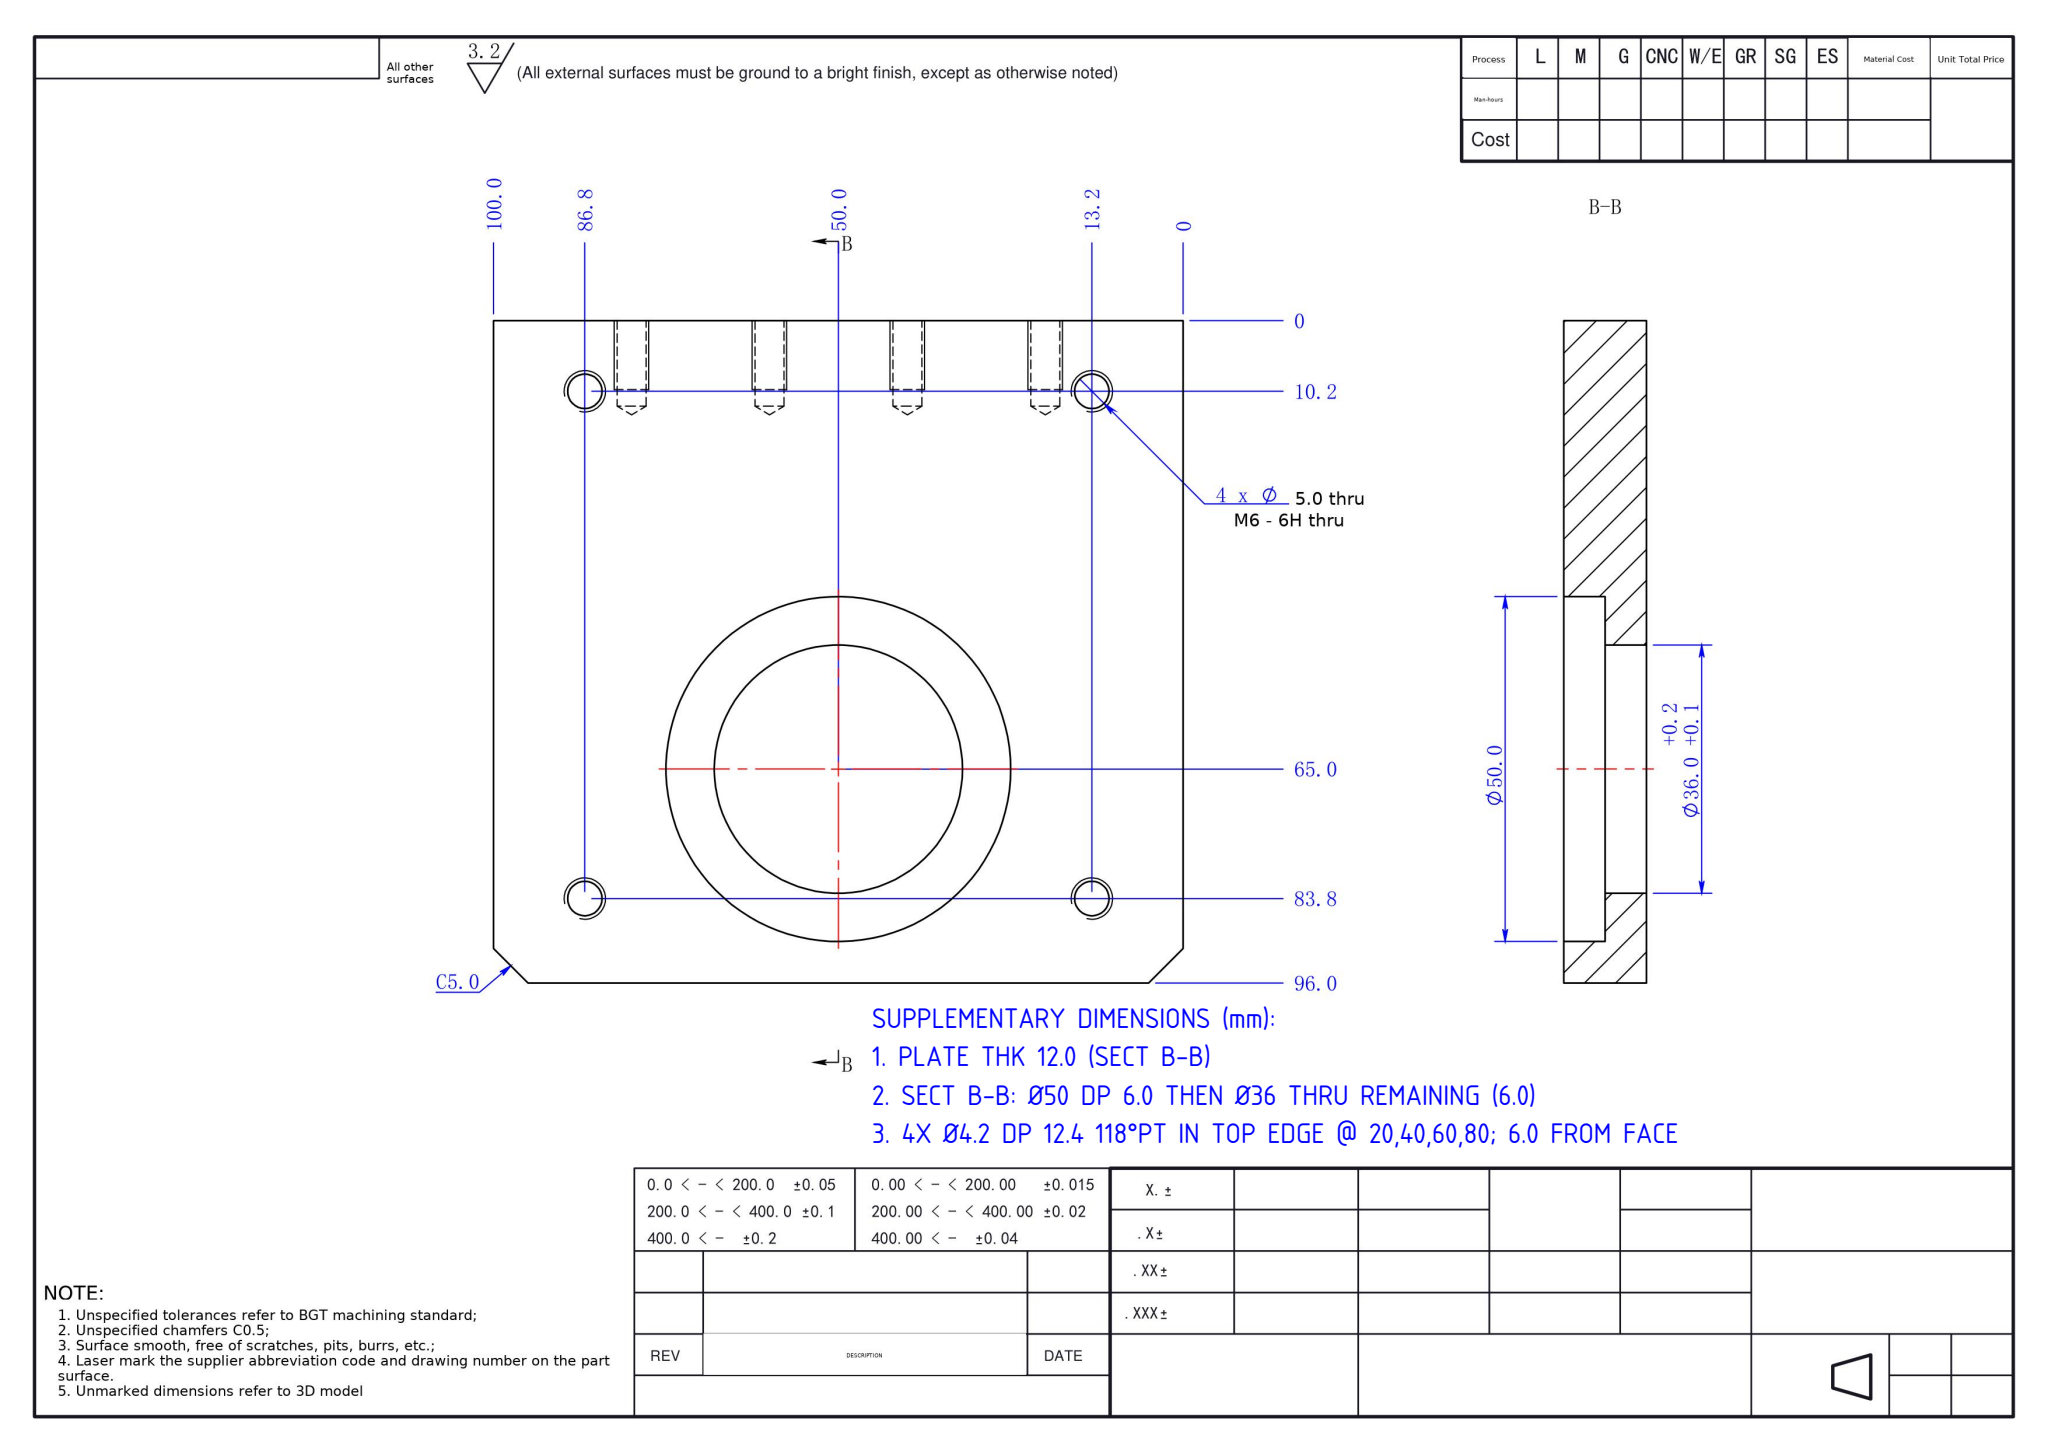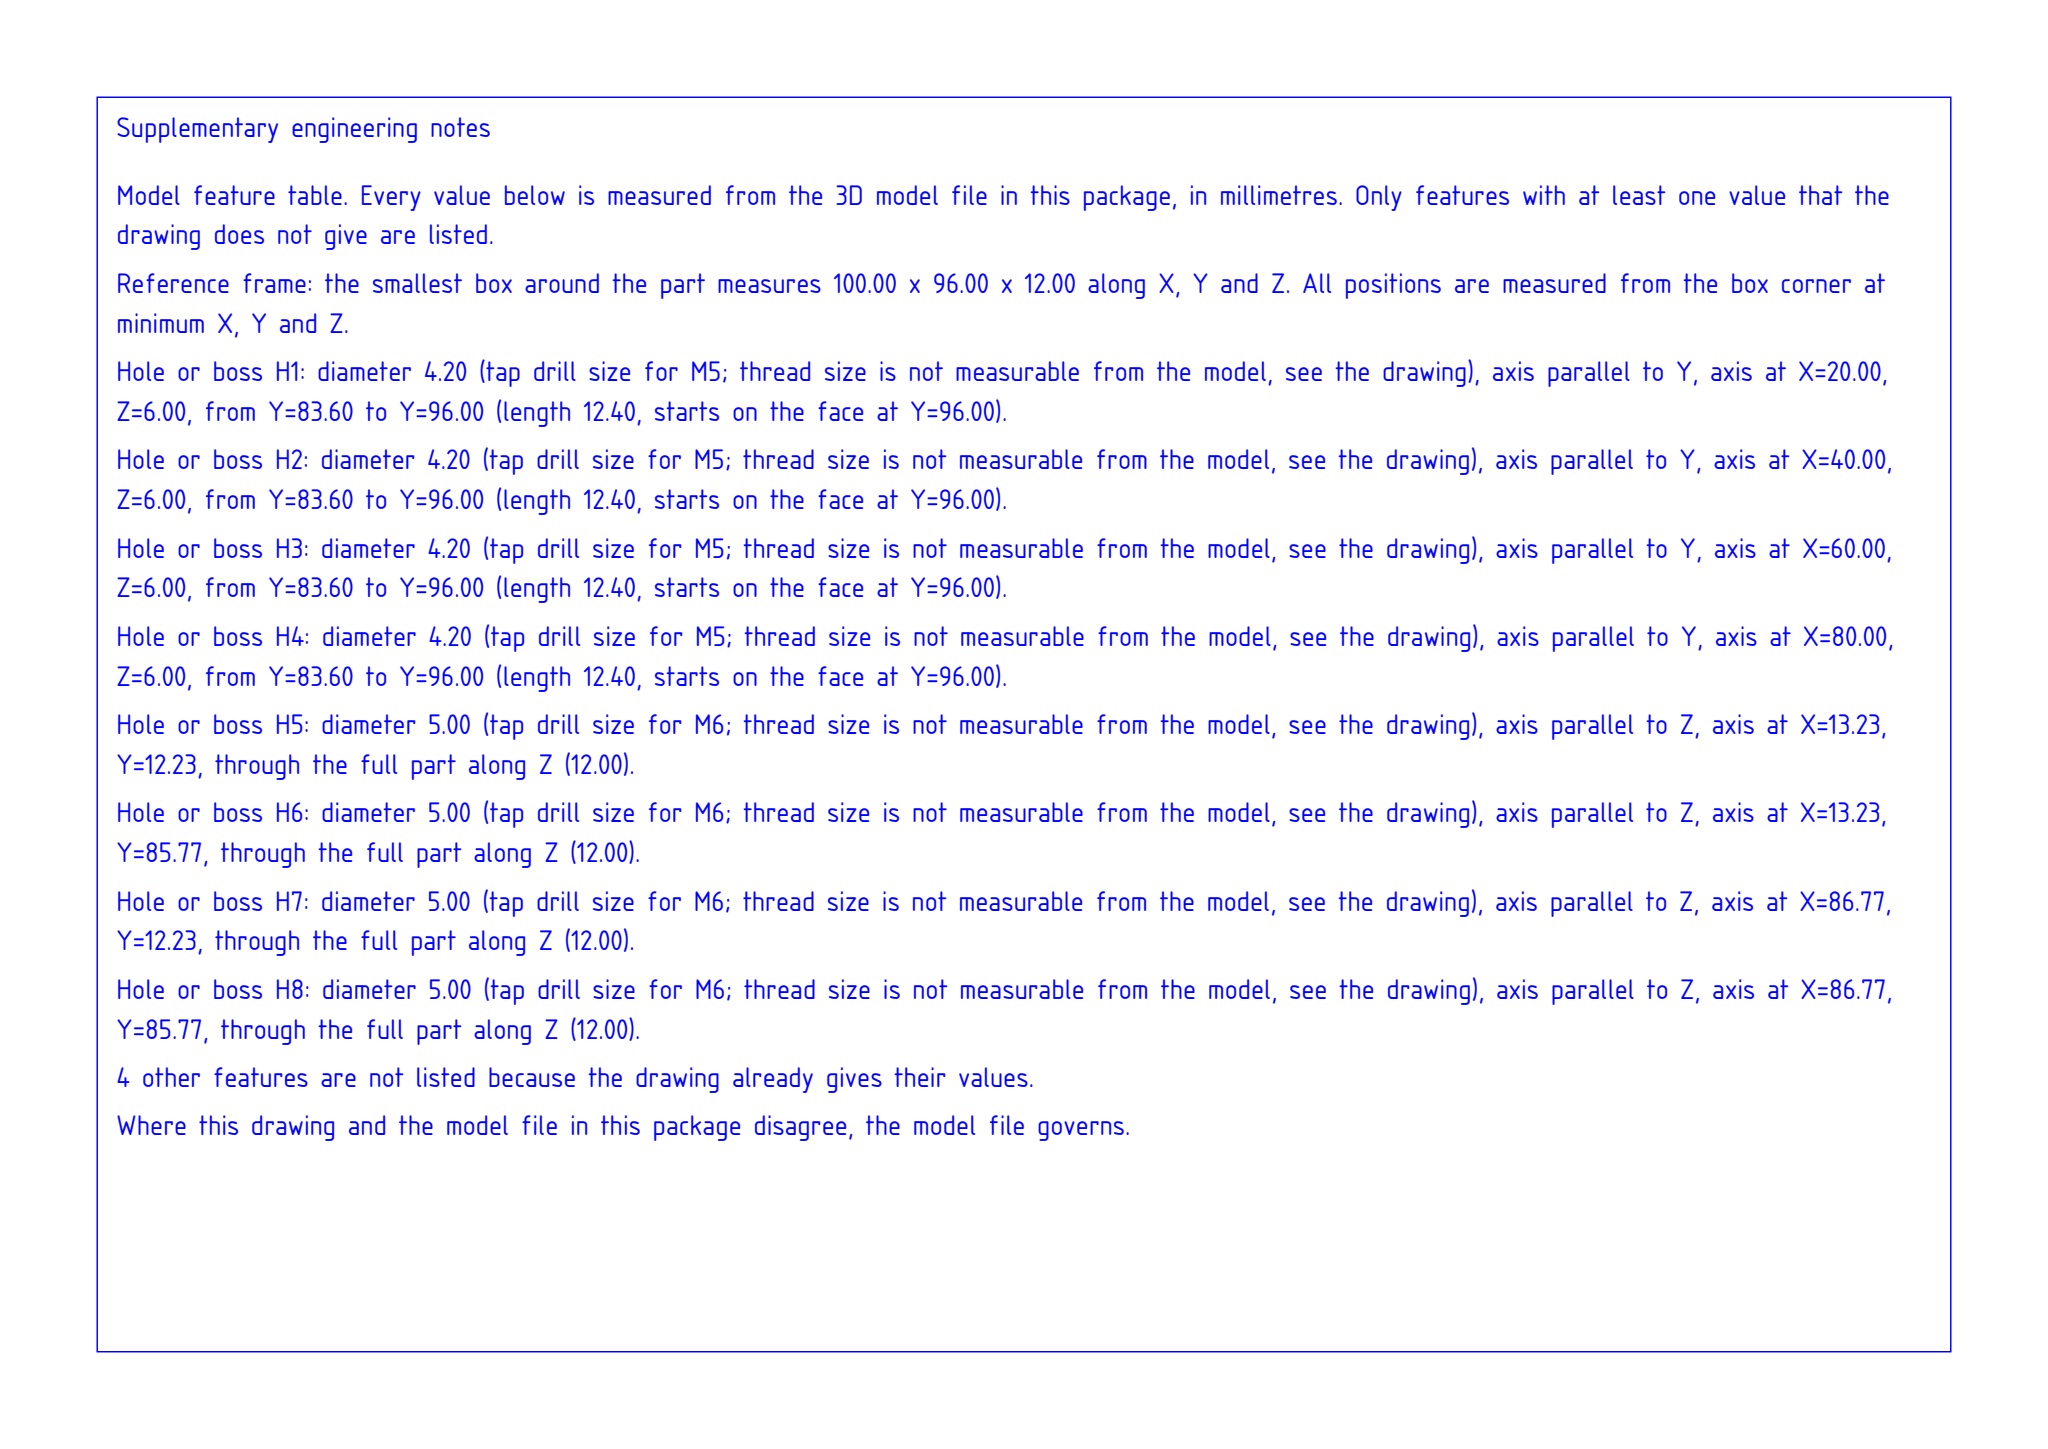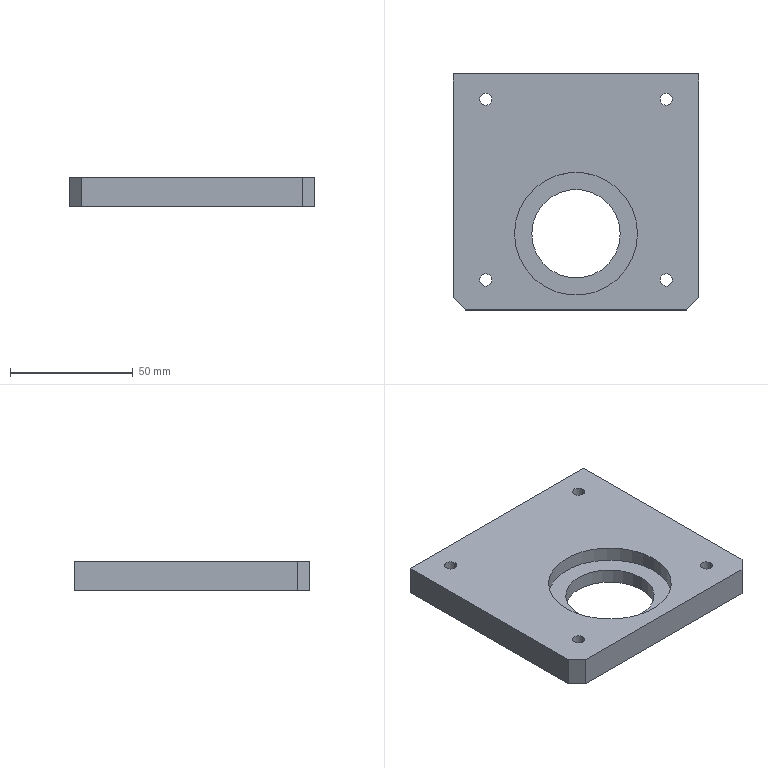Part | SolidWorks | mm | 1 solid | 37 faces | box 100 x 96 x 12 mm | volume 95359 mm3 | cylinder 20 | plane 9 | cone 8 | commonest cylinder face diameters 4.2 x8 5 x8 50 x2 36 x2
build123d program:
from build123d import *

# Parameters (mm, degrees)
SKETCH1_W             = 100
SKETCH1_H             = 96
BOSS_EXTRUDE1_DEPTH   = 12
SKETCH2_R             = 18
CUT_EXTRUDE1_DEPTH    = 140.14
CHAMFER1_SIZE         = 5
M6_TAPPED_HOLE1_D     = 5
SKETCH5_R             = 25
CUT_EXTRUDE2_DEPTH    = 6
M5_TAPPED_HOLE1_D     = 4.2
M5_TAPPED_HOLE1_DEPTH = 12.4
M5_TAPPED_HOLE1_TIP   = 1.262


with BuildPart() as part:
    # Sketch1 → Boss-Extrude1 (new body)
    with BuildSketch(Plane.XY):
        with Locations((50, 48)):
            Rectangle(SKETCH1_W, SKETCH1_H)
    extrude(amount=BOSS_EXTRUDE1_DEPTH)

    # Sketch2 → Cut-Extrude1 (cut, through all)
    with BuildSketch(Plane.XY.offset(12)):
        with Locations((50, 31)):
            Circle(SKETCH2_R)
    extrude(amount=-CUT_EXTRUDE1_DEPTH, mode=Mode.SUBTRACT)

    # Chamfer1
    chamfer1_edges = [part.edges().sort_by_distance(p)[0] for p in [
        (100, 0, 6),
        (0, 0, 6),
    ]]
    chamfer(chamfer1_edges, length=CHAMFER1_SIZE)

    # M6 Tapped Hole1 (through all)
    with Locations(Plane(origin=(0, 0, 0), x_dir=(-1, 0, 0), z_dir=(0, 0, -1))):
        with Locations((-86.77, 85.77), (-13.23, 85.77), (-13.23, 12.23), (-86.77, 12.23)):
            Hole(M6_TAPPED_HOLE1_D / 2)

    # Sketch5 → Cut-Extrude2 (cut)
    with BuildSketch(Plane.XY.offset(12)):
        with Locations((50, 31)):
            Circle(SKETCH5_R)
    extrude(amount=-CUT_EXTRUDE2_DEPTH, mode=Mode.SUBTRACT)

    # M5 Tapped Hole1
    with Locations(Plane(origin=(0, 96, 0), x_dir=(1, 0, 0), z_dir=(0, 1, 0))):
        with Locations((20, -6), (40, -6), (60, -6), (80, -6)):
            Hole(M5_TAPPED_HOLE1_D / 2, depth=M5_TAPPED_HOLE1_DEPTH)
            with Locations((0, 0, -(M5_TAPPED_HOLE1_DEPTH + M5_TAPPED_HOLE1_TIP / 2))):  # 118° drill point
                Cone(0, M5_TAPPED_HOLE1_D / 2, M5_TAPPED_HOLE1_TIP, mode=Mode.SUBTRACT)


solid = part.part